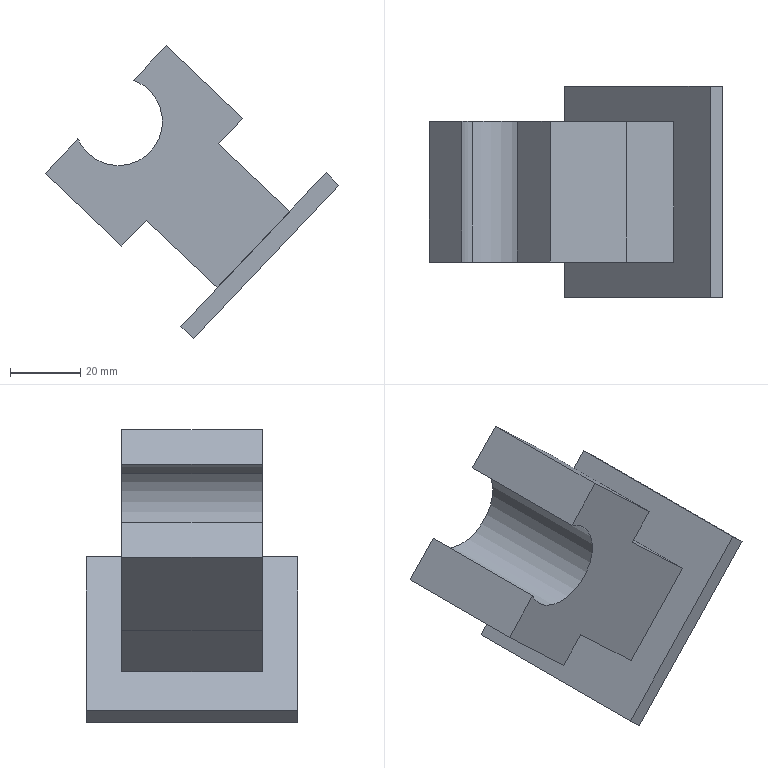Component | SolidWorks | 20mL - Glass Syringe-1_InjectionFixture-1 | 1 solid | 19 faces | box 83.45 x 60 x 83.15 mm | volume 96732 mm3 | plane 16 | cylinder 3 | commonest cylinder face diameters 25 x3
build123d program:
from build123d import *

# Parameters (mm, degrees)
BOSS_EXTRUDE1_START = -20
BOSS_EXTRUDE1_DEPTH = 40
BOSS_EXTRUDE2_DEPTH = 40
SKETCH4_W           = 60
SKETCH4_H           = 60
BOSS_EXTRUDE3_DEPTH = 5


with BuildPart() as part:
    # Sketch2 → Boss-Extrude1 (new body)
    with BuildSketch(Plane.XY.offset(BOSS_EXTRUDE1_START)):
        with BuildLine():
            Line((-21.937, -5), (-11.456, -5))
            ThreePointArc((-11.456, -5), (0, 12.5), (11.456, -5))
            Line((11.456, -5), (21.937, -5))
            ThreePointArc((21.937, -5), (0, 22.5), (-21.937, -5))
        make_face()
    extrude(amount=-BOSS_EXTRUDE1_DEPTH)

    # Sketch3 → Boss-Extrude2 (add)
    with BuildSketch(Plane.XY.offset(-20)):
        Polygon((15, 25.844), (15, 52.844), (-15, 52.844), (-15, 25.844), (-15, 25), (-25, 25), (-25, 20), (-25, -5), (-21.937, -5), (-17.95, 2.034), (-12.785, 12.264), (2.398, 17.259), (11.226, 13.398), (21.937, -5), (25, -5), (25, 20), (25, 25), (15, 25), align=None)
    extrude(amount=-BOSS_EXTRUDE2_DEPTH)

    # Sketch4 → Boss-Extrude3 (add)
    with BuildSketch(Plane(origin=(0, 52.844, 0), x_dir=(1, 0, 0), z_dir=(0, 1, 0))):
        with Locations((0, 40)):
            Rectangle(SKETCH4_W, SKETCH4_H)
    extrude(amount=BOSS_EXTRUDE3_DEPTH)


solid = part.part

# Placed as in the assembly
solid = solid.moved(Location((417.806, 1252, -1928.012), (90, 0, -133.462)))
STEP:
#1=CARTESIAN_POINT('',(15.996,50.079,-76.098));
#2=VERTEX_POINT('',#1);
#3=CARTESIAN_POINT('',(16.111,50.079,-76.263));
#4=VERTEX_POINT('',#3);
#5=CARTESIAN_POINT('',(16.449,50.079,-75.906));
#6=DIRECTION('',(0.,-1.,0.));
#7=DIRECTION('',(0.6879,0.,0.7258));
#8=AXIS2_PLACEMENT_3D('',#5,#6,#7);
#9=CIRCLE('',#8,0.4921);
#10=EDGE_CURVE('',#2,#4,#9,.T.);
#11=ORIENTED_EDGE('',*,*,#10,.T.);
#12=CARTESIAN_POINT('',(16.111,51.654,-76.263));
#13=VERTEX_POINT('',#12);
#14=CARTESIAN_POINT('',(16.111,50.079,-76.263));
#15=DIRECTION('',(-0.,1.,-0.));
#16=VECTOR('',#15,39.37);
#17=LINE('',#14,#16);
#18=EDGE_CURVE('',#4,#13,#17,.T.);
#19=ORIENTED_EDGE('',*,*,#18,.T.);
#20=CARTESIAN_POINT('',(15.996,51.654,-76.098));
#21=VERTEX_POINT('',#20);
#22=CARTESIAN_POINT('',(16.449,51.654,-75.906));
#23=DIRECTION('',(0.,-1.,0.));
#24=DIRECTION('',(0.6879,0.,0.7258));
#25=AXIS2_PLACEMENT_3D('',#22,#23,#24);
#26=CIRCLE('',#25,0.4921);
#27=EDGE_CURVE('',#21,#13,#26,.T.);
#28=ORIENTED_EDGE('',*,*,#27,.F.);
#29=CARTESIAN_POINT('',(15.996,50.079,-76.098));
#30=DIRECTION('',(-0.,1.,-0.));
#31=VECTOR('',#30,39.37);
#32=LINE('',#29,#31);
#33=EDGE_CURVE('',#2,#21,#32,.T.);
#34=ORIENTED_EDGE('',*,*,#33,.F.);
#35=EDGE_LOOP('',(#11,#19,#28,#34));
#36=FACE_OUTER_BOUND('',#35,.T.);
#37=CARTESIAN_POINT('',(16.449,50.079,-75.906));
#38=DIRECTION('',(-0.,1.,-0.));
#39=DIRECTION('',(0.6879,0.,0.7258));
#40=AXIS2_PLACEMENT_3D('',#37,#38,#39);
#41=CYLINDRICAL_SURFACE('',#40,0.4921);
#42=ADVANCED_FACE('',(#36),#41,.F.);
#43=ORIENTED_EDGE('',*,*,#18,.F.);
#44=CARTESIAN_POINT('',(16.788,50.079,-75.549));
#45=VERTEX_POINT('',#44);
#46=CARTESIAN_POINT('',(16.449,50.079,-75.906));
#47=DIRECTION('',(0.,-1.,0.));
#48=DIRECTION('',(0.6879,0.,0.7258));
#49=AXIS2_PLACEMENT_3D('',#46,#47,#48);
#50=CIRCLE('',#49,0.4921);
#51=EDGE_CURVE('',#4,#45,#50,.T.);
#52=ORIENTED_EDGE('',*,*,#51,.T.);
#53=CARTESIAN_POINT('',(16.788,51.654,-75.549));
#54=VERTEX_POINT('',#53);
#55=CARTESIAN_POINT('',(16.788,50.079,-75.549));
#56=DIRECTION('',(-0.,1.,-0.));
#57=VECTOR('',#56,39.37);
#58=LINE('',#55,#57);
#59=EDGE_CURVE('',#45,#54,#58,.T.);
#60=ORIENTED_EDGE('',*,*,#59,.T.);
#61=CARTESIAN_POINT('',(16.449,51.654,-75.906));
#62=DIRECTION('',(0.,-1.,0.));
#63=DIRECTION('',(0.6879,0.,0.7258));
#64=AXIS2_PLACEMENT_3D('',#61,#62,#63);
#65=CIRCLE('',#64,0.4921);
#66=EDGE_CURVE('',#13,#54,#65,.T.);
#67=ORIENTED_EDGE('',*,*,#66,.F.);
#68=EDGE_LOOP('',(#43,#52,#60,#67));
#69=FACE_OUTER_BOUND('',#68,.T.);
#70=CARTESIAN_POINT('',(16.449,50.079,-75.906));
#71=DIRECTION('',(-0.,1.,-0.));
#72=DIRECTION('',(0.6879,0.,0.7258));
#73=AXIS2_PLACEMENT_3D('',#70,#71,#72);
#74=CYLINDRICAL_SURFACE('',#73,0.4921);
#75=ADVANCED_FACE('',(#69),#74,.F.);
#76=CARTESIAN_POINT('',(16.616,51.654,-75.443));
#77=VERTEX_POINT('',#76);
#78=CARTESIAN_POINT('',(16.983,51.654,-75.056));
#79=VERTEX_POINT('',#78);
#80=CARTESIAN_POINT('',(16.616,51.654,-75.443));
#81=DIRECTION('',(0.6879,0.,0.7258));
#82=VECTOR('',#81,39.37);
#83=LINE('',#80,#82);
#84=EDGE_CURVE('',#77,#79,#83,.T.);
#85=ORIENTED_EDGE('',*,*,#84,.F.);
#86=CARTESIAN_POINT('',(16.616,50.079,-75.443));
#87=VERTEX_POINT('',#86);
#88=CARTESIAN_POINT('',(16.616,50.079,-75.443));
#89=DIRECTION('',(-0.,1.,-0.));
#90=VECTOR('',#89,39.37);
#91=LINE('',#88,#90);
#92=EDGE_CURVE('',#87,#77,#91,.T.);
#93=ORIENTED_EDGE('',*,*,#92,.F.);
#94=CARTESIAN_POINT('',(16.983,50.079,-75.056));
#95=VERTEX_POINT('',#94);
#96=CARTESIAN_POINT('',(16.616,50.079,-75.443));
#97=DIRECTION('',(0.6879,0.,0.7258));
#98=VECTOR('',#97,39.37);
#99=LINE('',#96,#98);
#100=EDGE_CURVE('',#87,#95,#99,.T.);
#101=ORIENTED_EDGE('',*,*,#100,.T.);
#102=CARTESIAN_POINT('',(16.983,50.079,-75.056));
#103=DIRECTION('',(-0.,1.,-0.));
#104=VECTOR('',#103,39.37);
#105=LINE('',#102,#104);
#106=EDGE_CURVE('',#95,#79,#105,.T.);
#107=ORIENTED_EDGE('',*,*,#106,.T.);
#108=EDGE_LOOP('',(#85,#93,#101,#107));
#109=FACE_OUTER_BOUND('',#108,.T.);
#110=CARTESIAN_POINT('',(16.616,50.079,-75.443));
#111=DIRECTION('',(-0.7258,-0.,0.6879));
#112=DIRECTION('',(0.,-1.,0.));
#113=AXIS2_PLACEMENT_3D('',#110,#111,#112);
#114=PLANE('',#113);
#115=ADVANCED_FACE('',(#109),#114,.T.);
#116=ORIENTED_EDGE('',*,*,#59,.F.);
#117=CARTESIAN_POINT('',(16.449,50.079,-75.906));
#118=DIRECTION('',(0.,-1.,0.));
#119=DIRECTION('',(0.6879,0.,0.7258));
#120=AXIS2_PLACEMENT_3D('',#117,#118,#119);
#121=CIRCLE('',#120,0.4921);
#122=EDGE_CURVE('',#45,#87,#121,.T.);
#123=ORIENTED_EDGE('',*,*,#122,.T.);
#124=ORIENTED_EDGE('',*,*,#92,.T.);
#125=CARTESIAN_POINT('',(16.449,51.654,-75.906));
#126=DIRECTION('',(0.,-1.,0.));
#127=DIRECTION('',(0.6879,0.,0.7258));
#128=AXIS2_PLACEMENT_3D('',#125,#126,#127);
#129=CIRCLE('',#128,0.4921);
#130=EDGE_CURVE('',#54,#77,#129,.T.);
#131=ORIENTED_EDGE('',*,*,#130,.F.);
#132=EDGE_LOOP('',(#116,#123,#124,#131));
#133=FACE_OUTER_BOUND('',#132,.T.);
#134=CARTESIAN_POINT('',(16.449,50.079,-75.906));
#135=DIRECTION('',(-0.,1.,-0.));
#136=DIRECTION('',(0.6879,0.,0.7258));
#137=AXIS2_PLACEMENT_3D('',#134,#135,#136);
#138=CYLINDRICAL_SURFACE('',#137,0.4921);
#139=ADVANCED_FACE('',(#133),#138,.F.);
#140=CARTESIAN_POINT('',(15.629,51.654,-76.485));
#141=VERTEX_POINT('',#140);
#142=CARTESIAN_POINT('',(15.712,51.654,-76.397));
#143=DIRECTION('',(0.6879,0.,0.7258));
#144=VECTOR('',#143,39.37);
#145=LINE('',#142,#144);
#146=EDGE_CURVE('',#141,#21,#145,.T.);
#147=ORIENTED_EDGE('',*,*,#146,.F.);
#148=CARTESIAN_POINT('',(15.629,50.079,-76.485));
#149=VERTEX_POINT('',#148);
#150=CARTESIAN_POINT('',(15.629,50.079,-76.485));
#151=DIRECTION('',(-0.,1.,-0.));
#152=VECTOR('',#151,39.37);
#153=LINE('',#150,#152);
#154=EDGE_CURVE('',#149,#141,#153,.T.);
#155=ORIENTED_EDGE('',*,*,#154,.F.);
#156=CARTESIAN_POINT('',(15.712,50.079,-76.397));
#157=DIRECTION('',(0.6879,0.,0.7258));
#158=VECTOR('',#157,39.37);
#159=LINE('',#156,#158);
#160=EDGE_CURVE('',#149,#2,#159,.T.);
#161=ORIENTED_EDGE('',*,*,#160,.T.);
#162=ORIENTED_EDGE('',*,*,#33,.T.);
#163=EDGE_LOOP('',(#147,#155,#161,#162));
#164=FACE_OUTER_BOUND('',#163,.T.);
#165=CARTESIAN_POINT('',(15.712,50.079,-76.397));
#166=DIRECTION('',(-0.7258,-0.,0.6879));
#167=DIRECTION('',(0.,-1.,0.));
#168=AXIS2_PLACEMENT_3D('',#165,#166,#167);
#169=PLANE('',#168);
#170=ADVANCED_FACE('',(#164),#169,.T.);
#171=ORIENTED_EDGE('',*,*,#160,.F.);
#172=CARTESIAN_POINT('',(16.486,50.079,-77.297));
#173=VERTEX_POINT('',#172);
#174=CARTESIAN_POINT('',(16.486,50.079,-77.297));
#175=DIRECTION('',(-0.7258,-0.,0.6879));
#176=VECTOR('',#175,39.37);
#177=LINE('',#174,#176);
#178=EDGE_CURVE('',#173,#149,#177,.T.);
#179=ORIENTED_EDGE('',*,*,#178,.F.);
#180=CARTESIAN_POINT('',(16.757,50.079,-77.012));
#181=VERTEX_POINT('',#180);
#182=CARTESIAN_POINT('',(16.486,50.079,-77.297));
#183=DIRECTION('',(-0.6879,-0.,-0.7258));
#184=VECTOR('',#183,39.37);
#185=LINE('',#182,#184);
#186=EDGE_CURVE('',#181,#173,#185,.T.);
#187=ORIENTED_EDGE('',*,*,#186,.F.);
#188=CARTESIAN_POINT('',(17.553,50.079,-77.766));
#189=VERTEX_POINT('',#188);
#190=CARTESIAN_POINT('',(17.553,50.079,-77.766));
#191=DIRECTION('',(-0.7258,-0.,0.6879));
#192=VECTOR('',#191,39.37);
#193=LINE('',#190,#192);
#194=EDGE_CURVE('',#189,#181,#193,.T.);
#195=ORIENTED_EDGE('',*,*,#194,.F.);
#196=CARTESIAN_POINT('',(18.365,50.079,-76.908));
#197=VERTEX_POINT('',#196);
#198=CARTESIAN_POINT('',(18.365,50.079,-76.908));
#199=DIRECTION('',(-0.6879,-0.,-0.7258));
#200=VECTOR('',#199,39.37);
#201=LINE('',#198,#200);
#202=EDGE_CURVE('',#197,#189,#201,.T.);
#203=ORIENTED_EDGE('',*,*,#202,.F.);
#204=CARTESIAN_POINT('',(17.57,50.079,-76.154));
#205=VERTEX_POINT('',#204);
#206=CARTESIAN_POINT('',(17.594,50.079,-76.177));
#207=DIRECTION('',(0.7258,0.,-0.6879));
#208=VECTOR('',#207,39.37);
#209=LINE('',#206,#208);
#210=EDGE_CURVE('',#205,#197,#209,.T.);
#211=ORIENTED_EDGE('',*,*,#210,.F.);
#212=CARTESIAN_POINT('',(17.84,50.079,-75.869));
#213=VERTEX_POINT('',#212);
#214=CARTESIAN_POINT('',(17.57,50.079,-76.154));
#215=DIRECTION('',(-0.6879,-0.,-0.7258));
#216=VECTOR('',#215,39.37);
#217=LINE('',#214,#216);
#218=EDGE_CURVE('',#213,#205,#217,.T.);
#219=ORIENTED_EDGE('',*,*,#218,.F.);
#220=CARTESIAN_POINT('',(16.983,50.079,-75.056));
#221=DIRECTION('',(0.7258,0.,-0.6879));
#222=VECTOR('',#221,39.37);
#223=LINE('',#220,#222);
#224=EDGE_CURVE('',#95,#213,#223,.T.);
#225=ORIENTED_EDGE('',*,*,#224,.F.);
#226=ORIENTED_EDGE('',*,*,#100,.F.);
#227=ORIENTED_EDGE('',*,*,#122,.F.);
#228=ORIENTED_EDGE('',*,*,#51,.F.);
#229=ORIENTED_EDGE('',*,*,#10,.F.);
#230=EDGE_LOOP('',(#171,#179,#187,#195,#203,#211,#219,#225,#226,#227,#228,#229));
#231=FACE_OUTER_BOUND('',#230,.T.);
#232=CARTESIAN_POINT('',(16.449,50.079,-75.906));
#233=DIRECTION('',(-0.,1.,-0.));
#234=DIRECTION('',(0.6879,0.,0.7258));
#235=AXIS2_PLACEMENT_3D('',#232,#233,#234);
#236=PLANE('',#235);
#237=ADVANCED_FACE('',(#231),#236,.F.);
#238=ORIENTED_EDGE('',*,*,#84,.T.);
#239=CARTESIAN_POINT('',(17.84,51.654,-75.869));
#240=VERTEX_POINT('',#239);
#241=CARTESIAN_POINT('',(17.84,51.654,-75.869));
#242=DIRECTION('',(0.7258,0.,-0.6879));
#243=VECTOR('',#242,39.37);
#244=LINE('',#241,#243);
#245=EDGE_CURVE('',#79,#240,#244,.T.);
#246=ORIENTED_EDGE('',*,*,#245,.T.);
#247=CARTESIAN_POINT('',(17.57,51.654,-76.154));
#248=VERTEX_POINT('',#247);
#249=CARTESIAN_POINT('',(17.57,51.654,-76.154));
#250=DIRECTION('',(-0.6879,-0.,-0.7258));
#251=VECTOR('',#250,39.37);
#252=LINE('',#249,#251);
#253=EDGE_CURVE('',#240,#248,#252,.T.);
#254=ORIENTED_EDGE('',*,*,#253,.T.);
#255=CARTESIAN_POINT('',(18.365,51.654,-76.908));
#256=VERTEX_POINT('',#255);
#257=CARTESIAN_POINT('',(17.594,51.654,-76.177));
#258=DIRECTION('',(0.7258,0.,-0.6879));
#259=VECTOR('',#258,39.37);
#260=LINE('',#257,#259);
#261=EDGE_CURVE('',#248,#256,#260,.T.);
#262=ORIENTED_EDGE('',*,*,#261,.T.);
#263=CARTESIAN_POINT('',(17.553,51.654,-77.766));
#264=VERTEX_POINT('',#263);
#265=CARTESIAN_POINT('',(18.365,51.654,-76.908));
#266=DIRECTION('',(-0.6879,-0.,-0.7258));
#267=VECTOR('',#266,39.37);
#268=LINE('',#265,#267);
#269=EDGE_CURVE('',#256,#264,#268,.T.);
#270=ORIENTED_EDGE('',*,*,#269,.T.);
#271=CARTESIAN_POINT('',(16.757,51.654,-77.012));
#272=VERTEX_POINT('',#271);
#273=CARTESIAN_POINT('',(16.781,51.654,-77.035));
#274=DIRECTION('',(-0.7258,-0.,0.6879));
#275=VECTOR('',#274,39.37);
#276=LINE('',#273,#275);
#277=EDGE_CURVE('',#264,#272,#276,.T.);
#278=ORIENTED_EDGE('',*,*,#277,.T.);
#279=CARTESIAN_POINT('',(16.486,51.654,-77.297));
#280=VERTEX_POINT('',#279);
#281=CARTESIAN_POINT('',(16.486,51.654,-77.297));
#282=DIRECTION('',(-0.6879,-0.,-0.7258));
#283=VECTOR('',#282,39.37);
#284=LINE('',#281,#283);
#285=EDGE_CURVE('',#272,#280,#284,.T.);
#286=ORIENTED_EDGE('',*,*,#285,.T.);
#287=CARTESIAN_POINT('',(15.629,51.654,-76.485));
#288=DIRECTION('',(-0.7258,-0.,0.6879));
#289=VECTOR('',#288,39.37);
#290=LINE('',#287,#289);
#291=EDGE_CURVE('',#280,#141,#290,.T.);
#292=ORIENTED_EDGE('',*,*,#291,.T.);
#293=ORIENTED_EDGE('',*,*,#146,.T.);
#294=ORIENTED_EDGE('',*,*,#27,.T.);
#295=ORIENTED_EDGE('',*,*,#66,.T.);
#296=ORIENTED_EDGE('',*,*,#130,.T.);
#297=EDGE_LOOP('',(#238,#246,#254,#262,#270,#278,#286,#292,#293,#294,#295,#296));
#298=FACE_OUTER_BOUND('',#297,.T.);
#299=CARTESIAN_POINT('',(16.449,51.654,-75.906));
#300=DIRECTION('',(-0.,1.,-0.));
#301=DIRECTION('',(0.6879,0.,0.7258));
#302=AXIS2_PLACEMENT_3D('',#299,#300,#301);
#303=PLANE('',#302);
#304=ADVANCED_FACE('',(#298),#303,.T.);
#305=ORIENTED_EDGE('',*,*,#291,.F.);
#306=CARTESIAN_POINT('',(16.486,50.079,-77.297));
#307=DIRECTION('',(-0.,1.,-0.));
#308=VECTOR('',#307,39.37);
#309=LINE('',#306,#308);
#310=EDGE_CURVE('',#173,#280,#309,.T.);
#311=ORIENTED_EDGE('',*,*,#310,.F.);
#312=ORIENTED_EDGE('',*,*,#178,.T.);
#313=ORIENTED_EDGE('',*,*,#154,.T.);
#314=EDGE_LOOP('',(#305,#311,#312,#313));
#315=FACE_OUTER_BOUND('',#314,.T.);
#316=CARTESIAN_POINT('',(15.629,50.079,-76.485));
#317=DIRECTION('',(-0.6879,-0.,-0.7258));
#318=DIRECTION('',(-0.,1.,-0.));
#319=AXIS2_PLACEMENT_3D('',#316,#317,#318);
#320=PLANE('',#319);
#321=ADVANCED_FACE('',(#315),#320,.T.);
#322=ORIENTED_EDGE('',*,*,#285,.F.);
#323=CARTESIAN_POINT('',(16.757,50.079,-77.012));
#324=DIRECTION('',(-0.,1.,-0.));
#325=VECTOR('',#324,39.37);
#326=LINE('',#323,#325);
#327=EDGE_CURVE('',#181,#272,#326,.T.);
#328=ORIENTED_EDGE('',*,*,#327,.F.);
#329=ORIENTED_EDGE('',*,*,#186,.T.);
#330=ORIENTED_EDGE('',*,*,#310,.T.);
#331=EDGE_LOOP('',(#322,#328,#329,#330));
#332=FACE_OUTER_BOUND('',#331,.T.);
#333=CARTESIAN_POINT('',(16.486,50.079,-77.297));
#334=DIRECTION('',(0.7258,0.,-0.6879));
#335=DIRECTION('',(-0.,1.,-0.));
#336=AXIS2_PLACEMENT_3D('',#333,#334,#335);
#337=PLANE('',#336);
#338=ADVANCED_FACE('',(#332),#337,.T.);
#339=ORIENTED_EDGE('',*,*,#277,.F.);
#340=CARTESIAN_POINT('',(17.553,50.079,-77.766));
#341=DIRECTION('',(-0.,1.,-0.));
#342=VECTOR('',#341,39.37);
#343=LINE('',#340,#342);
#344=EDGE_CURVE('',#189,#264,#343,.T.);
#345=ORIENTED_EDGE('',*,*,#344,.F.);
#346=ORIENTED_EDGE('',*,*,#194,.T.);
#347=ORIENTED_EDGE('',*,*,#327,.T.);
#348=EDGE_LOOP('',(#339,#345,#346,#347));
#349=FACE_OUTER_BOUND('',#348,.T.);
#350=CARTESIAN_POINT('',(16.781,50.079,-77.035));
#351=DIRECTION('',(-0.6879,-0.,-0.7258));
#352=DIRECTION('',(-0.,1.,-0.));
#353=AXIS2_PLACEMENT_3D('',#350,#351,#352);
#354=PLANE('',#353);
#355=ADVANCED_FACE('',(#349),#354,.T.);
#356=ORIENTED_EDGE('',*,*,#261,.F.);
#357=CARTESIAN_POINT('',(17.57,50.079,-76.154));
#358=DIRECTION('',(-0.,1.,-0.));
#359=VECTOR('',#358,39.37);
#360=LINE('',#357,#359);
#361=EDGE_CURVE('',#205,#248,#360,.T.);
#362=ORIENTED_EDGE('',*,*,#361,.F.);
#363=ORIENTED_EDGE('',*,*,#210,.T.);
#364=CARTESIAN_POINT('',(18.365,50.079,-76.908));
#365=DIRECTION('',(-0.,1.,-0.));
#366=VECTOR('',#365,39.37);
#367=LINE('',#364,#366);
#368=EDGE_CURVE('',#197,#256,#367,.T.);
#369=ORIENTED_EDGE('',*,*,#368,.T.);
#370=EDGE_LOOP('',(#356,#362,#363,#369));
#371=FACE_OUTER_BOUND('',#370,.T.);
#372=CARTESIAN_POINT('',(17.594,50.079,-76.177));
#373=DIRECTION('',(0.6879,0.,0.7258));
#374=DIRECTION('',(0.,-1.,0.));
#375=AXIS2_PLACEMENT_3D('',#372,#373,#374);
#376=PLANE('',#375);
#377=ADVANCED_FACE('',(#371),#376,.T.);
#378=ORIENTED_EDGE('',*,*,#253,.F.);
#379=CARTESIAN_POINT('',(17.84,50.079,-75.869));
#380=DIRECTION('',(-0.,1.,-0.));
#381=VECTOR('',#380,39.37);
#382=LINE('',#379,#381);
#383=EDGE_CURVE('',#213,#240,#382,.T.);
#384=ORIENTED_EDGE('',*,*,#383,.F.);
#385=ORIENTED_EDGE('',*,*,#218,.T.);
#386=ORIENTED_EDGE('',*,*,#361,.T.);
#387=EDGE_LOOP('',(#378,#384,#385,#386));
#388=FACE_OUTER_BOUND('',#387,.T.);
#389=CARTESIAN_POINT('',(17.57,50.079,-76.154));
#390=DIRECTION('',(0.7258,0.,-0.6879));
#391=DIRECTION('',(-0.,1.,-0.));
#392=AXIS2_PLACEMENT_3D('',#389,#390,#391);
#393=PLANE('',#392);
#394=ADVANCED_FACE('',(#388),#393,.T.);
#395=ORIENTED_EDGE('',*,*,#245,.F.);
#396=ORIENTED_EDGE('',*,*,#106,.F.);
#397=ORIENTED_EDGE('',*,*,#224,.T.);
#398=ORIENTED_EDGE('',*,*,#383,.T.);
#399=EDGE_LOOP('',(#395,#396,#397,#398));
#400=FACE_OUTER_BOUND('',#399,.T.);
#401=CARTESIAN_POINT('',(17.84,50.079,-75.869));
#402=DIRECTION('',(0.6879,0.,0.7258));
#403=DIRECTION('',(0.,-1.,0.));
#404=AXIS2_PLACEMENT_3D('',#401,#402,#403);
#405=PLANE('',#404);
#406=ADVANCED_FACE('',(#400),#405,.T.);
#407=CARTESIAN_POINT('',(17.147,49.685,-78.194));
#408=VERTEX_POINT('',#407);
#409=CARTESIAN_POINT('',(17.147,52.047,-78.194));
#410=VERTEX_POINT('',#409);
#411=CARTESIAN_POINT('',(17.147,49.685,-78.194));
#412=DIRECTION('',(-0.,1.,-0.));
#413=VECTOR('',#412,39.37);
#414=LINE('',#411,#413);
#415=EDGE_CURVE('',#408,#410,#414,.T.);
#416=ORIENTED_EDGE('',*,*,#415,.F.);
#417=CARTESIAN_POINT('',(18.772,49.685,-76.48));
#418=VERTEX_POINT('',#417);
#419=CARTESIAN_POINT('',(18.772,49.685,-76.48));
#420=DIRECTION('',(-0.6879,-0.,-0.7258));
#421=VECTOR('',#420,39.37);
#422=LINE('',#419,#421);
#423=EDGE_CURVE('',#418,#408,#422,.T.);
#424=ORIENTED_EDGE('',*,*,#423,.F.);
#425=CARTESIAN_POINT('',(18.772,52.047,-76.48));
#426=VERTEX_POINT('',#425);
#427=CARTESIAN_POINT('',(18.772,49.685,-76.48));
#428=DIRECTION('',(0.,-1.,0.));
#429=VECTOR('',#428,39.37);
#430=LINE('',#427,#429);
#431=EDGE_CURVE('',#426,#418,#430,.T.);
#432=ORIENTED_EDGE('',*,*,#431,.F.);
#433=CARTESIAN_POINT('',(18.772,52.047,-76.48));
#434=DIRECTION('',(0.6879,0.,0.7258));
#435=VECTOR('',#434,39.37);
#436=LINE('',#433,#435);
#437=EDGE_CURVE('',#410,#426,#436,.T.);
#438=ORIENTED_EDGE('',*,*,#437,.F.);
#439=EDGE_LOOP('',(#416,#424,#432,#438));
#440=FACE_OUTER_BOUND('',#439,.T.);
#441=ORIENTED_EDGE('',*,*,#269,.F.);
#442=ORIENTED_EDGE('',*,*,#368,.F.);
#443=ORIENTED_EDGE('',*,*,#202,.T.);
#444=ORIENTED_EDGE('',*,*,#344,.T.);
#445=EDGE_LOOP('',(#441,#442,#443,#444));
#446=FACE_BOUND('',#445,.T.);
#447=CARTESIAN_POINT('',(17.959,52.441,-77.337));
#448=DIRECTION('',(-0.7258,-0.,0.6879));
#449=DIRECTION('',(0.6879,0.,0.7258));
#450=AXIS2_PLACEMENT_3D('',#447,#448,#449);
#451=PLANE('',#450);
#452=ADVANCED_FACE('',(#440,#446),#451,.T.);
#453=ORIENTED_EDGE('',*,*,#415,.T.);
#454=CARTESIAN_POINT('',(17.29,52.047,-78.33));
#455=VERTEX_POINT('',#454);
#456=CARTESIAN_POINT('',(17.29,52.047,-78.33));
#457=DIRECTION('',(-0.7258,-0.,0.6879));
#458=VECTOR('',#457,39.37);
#459=LINE('',#456,#458);
#460=EDGE_CURVE('',#455,#410,#459,.T.);
#461=ORIENTED_EDGE('',*,*,#460,.F.);
#462=CARTESIAN_POINT('',(17.29,49.685,-78.33));
#463=VERTEX_POINT('',#462);
#464=CARTESIAN_POINT('',(17.29,49.685,-78.33));
#465=DIRECTION('',(-0.,1.,-0.));
#466=VECTOR('',#465,39.37);
#467=LINE('',#464,#466);
#468=EDGE_CURVE('',#463,#455,#467,.T.);
#469=ORIENTED_EDGE('',*,*,#468,.F.);
#470=CARTESIAN_POINT('',(17.29,49.685,-78.33));
#471=DIRECTION('',(-0.7258,-0.,0.6879));
#472=VECTOR('',#471,39.37);
#473=LINE('',#470,#472);
#474=EDGE_CURVE('',#463,#408,#473,.T.);
#475=ORIENTED_EDGE('',*,*,#474,.T.);
#476=EDGE_LOOP('',(#453,#461,#469,#475));
#477=FACE_OUTER_BOUND('',#476,.T.);
#478=CARTESIAN_POINT('',(17.29,49.685,-78.33));
#479=DIRECTION('',(0.6879,0.,0.7258));
#480=DIRECTION('',(0.7258,0.,-0.6879));
#481=AXIS2_PLACEMENT_3D('',#478,#479,#480);
#482=PLANE('',#481);
#483=ADVANCED_FACE('',(#477),#482,.F.);
#484=ORIENTED_EDGE('',*,*,#437,.T.);
#485=CARTESIAN_POINT('',(18.914,52.047,-76.615));
#486=VERTEX_POINT('',#485);
#487=CARTESIAN_POINT('',(18.914,52.047,-76.615));
#488=DIRECTION('',(-0.7258,-0.,0.6879));
#489=VECTOR('',#488,39.37);
#490=LINE('',#487,#489);
#491=EDGE_CURVE('',#486,#426,#490,.T.);
#492=ORIENTED_EDGE('',*,*,#491,.F.);
#493=CARTESIAN_POINT('',(18.914,52.047,-76.615));
#494=DIRECTION('',(0.6879,0.,0.7258));
#495=VECTOR('',#494,39.37);
#496=LINE('',#493,#495);
#497=EDGE_CURVE('',#455,#486,#496,.T.);
#498=ORIENTED_EDGE('',*,*,#497,.F.);
#499=ORIENTED_EDGE('',*,*,#460,.T.);
#500=EDGE_LOOP('',(#484,#492,#498,#499));
#501=FACE_OUTER_BOUND('',#500,.T.);
#502=CARTESIAN_POINT('',(18.914,52.047,-76.615));
#503=DIRECTION('',(0.,-1.,0.));
#504=DIRECTION('',(-0.6879,-0.,-0.7258));
#505=AXIS2_PLACEMENT_3D('',#502,#503,#504);
#506=PLANE('',#505);
#507=ADVANCED_FACE('',(#501),#506,.F.);
#508=ORIENTED_EDGE('',*,*,#431,.T.);
#509=CARTESIAN_POINT('',(18.914,49.685,-76.615));
#510=VERTEX_POINT('',#509);
#511=CARTESIAN_POINT('',(18.914,49.685,-76.615));
#512=DIRECTION('',(-0.7258,-0.,0.6879));
#513=VECTOR('',#512,39.37);
#514=LINE('',#511,#513);
#515=EDGE_CURVE('',#510,#418,#514,.T.);
#516=ORIENTED_EDGE('',*,*,#515,.F.);
#517=CARTESIAN_POINT('',(18.914,49.685,-76.615));
#518=DIRECTION('',(0.,-1.,0.));
#519=VECTOR('',#518,39.37);
#520=LINE('',#517,#519);
#521=EDGE_CURVE('',#486,#510,#520,.T.);
#522=ORIENTED_EDGE('',*,*,#521,.F.);
#523=ORIENTED_EDGE('',*,*,#491,.T.);
#524=EDGE_LOOP('',(#508,#516,#522,#523));
#525=FACE_OUTER_BOUND('',#524,.T.);
#526=CARTESIAN_POINT('',(18.914,49.685,-76.615));
#527=DIRECTION('',(-0.6879,-0.,-0.7258));
#528=DIRECTION('',(-0.7258,-0.,0.6879));
#529=AXIS2_PLACEMENT_3D('',#526,#527,#528);
#530=PLANE('',#529);
#531=ADVANCED_FACE('',(#525),#530,.F.);
#532=ORIENTED_EDGE('',*,*,#423,.T.);
#533=ORIENTED_EDGE('',*,*,#474,.F.);
#534=CARTESIAN_POINT('',(18.914,49.685,-76.615));
#535=DIRECTION('',(-0.6879,-0.,-0.7258));
#536=VECTOR('',#535,39.37);
#537=LINE('',#534,#536);
#538=EDGE_CURVE('',#510,#463,#537,.T.);
#539=ORIENTED_EDGE('',*,*,#538,.F.);
#540=ORIENTED_EDGE('',*,*,#515,.T.);
#541=EDGE_LOOP('',(#532,#533,#539,#540));
#542=FACE_OUTER_BOUND('',#541,.T.);
#543=CARTESIAN_POINT('',(18.914,49.685,-76.615));
#544=DIRECTION('',(-0.,1.,0.));
#545=DIRECTION('',(0.6879,0.,0.7258));
#546=AXIS2_PLACEMENT_3D('',#543,#544,#545);
#547=PLANE('',#546);
#548=ADVANCED_FACE('',(#542),#547,.F.);
#549=ORIENTED_EDGE('',*,*,#468,.T.);
#550=ORIENTED_EDGE('',*,*,#497,.T.);
#551=ORIENTED_EDGE('',*,*,#521,.T.);
#552=ORIENTED_EDGE('',*,*,#538,.T.);
#553=EDGE_LOOP('',(#549,#550,#551,#552));
#554=FACE_OUTER_BOUND('',#553,.T.);
#555=CARTESIAN_POINT('',(18.102,52.441,-77.472));
#556=DIRECTION('',(-0.7258,-0.,0.6879));
#557=DIRECTION('',(0.6879,0.,0.7258));
#558=AXIS2_PLACEMENT_3D('',#555,#556,#557);
#559=PLANE('',#558);
#560=ADVANCED_FACE('',(#554),#559,.F.);
#561=CLOSED_SHELL('',(#42,#75,#115,#139,#170,#237,#304,#321,#338,#355,#377,#394,#406,#452,#483,#507,#531,#548,#560));
#562=MANIFOLD_SOLID_BREP('',#561);
#563=CARTESIAN_POINT('',(0.,0.,0.));
#564=DIRECTION('',(0.,0.,1.));
#565=DIRECTION('',(1.,0.,0.));
#566=AXIS2_PLACEMENT_3D('',#563,#564,#565);
#567=(LENGTH_UNIT()NAMED_UNIT(*)SI_UNIT($,.METRE.));
#568=LENGTH_MEASURE_WITH_UNIT(LENGTH_MEASURE(0.0254),#567);
#569=DIMENSIONAL_EXPONENTS(1.,0.,0.,0.,0.,0.,0.);
#570=(CONVERSION_BASED_UNIT('',#568)LENGTH_UNIT()NAMED_UNIT(#569));
#571=UNCERTAINTY_MEASURE_WITH_UNIT(LENGTH_MEASURE(0.00001),#570,'','');
#572=(NAMED_UNIT(*)PLANE_ANGLE_UNIT()SI_UNIT($,.RADIAN.));
#573=(NAMED_UNIT(*)SI_UNIT($,.STERADIAN.)SOLID_ANGLE_UNIT());
#574=(GEOMETRIC_REPRESENTATION_CONTEXT(3)GLOBAL_UNCERTAINTY_ASSIGNED_CONTEXT((#571))GLOBAL_UNIT_ASSIGNED_CONTEXT((#570,#572,#573))REPRESENTATION_CONTEXT('',''));
#575=ADVANCED_BREP_SHAPE_REPRESENTATION('',(#562,#566),#574);
#576=COLOUR_RGB('',0.7922,0.8196,0.9333);
#577=FILL_AREA_STYLE_COLOUR('',#576);
#578=FILL_AREA_STYLE('',(#577));
#579=SURFACE_STYLE_FILL_AREA(#578);
#580=SURFACE_SIDE_STYLE('',(#579));
#581=SURFACE_STYLE_USAGE(.BOTH.,#580);
#582=PRESENTATION_STYLE_ASSIGNMENT((#581));
#583=STYLED_ITEM('',(#582),#562);
#584=PRESENTATION_LAYER_ASSIGNMENT('','',(#583));
#585=(LENGTH_UNIT()NAMED_UNIT(*)SI_UNIT($,.METRE.));
#586=LENGTH_MEASURE_WITH_UNIT(LENGTH_MEASURE(0.0254),#585);
#587=DIMENSIONAL_EXPONENTS(1.,0.,0.,0.,0.,0.,0.);
#588=(CONVERSION_BASED_UNIT('',#586)LENGTH_UNIT()NAMED_UNIT(#587));
#589=UNCERTAINTY_MEASURE_WITH_UNIT(LENGTH_MEASURE(0.00001),#588,'','');
#590=(NAMED_UNIT(*)PLANE_ANGLE_UNIT()SI_UNIT($,.RADIAN.));
#591=(NAMED_UNIT(*)SI_UNIT($,.STERADIAN.)SOLID_ANGLE_UNIT());
#592=(GEOMETRIC_REPRESENTATION_CONTEXT(3)GLOBAL_UNCERTAINTY_ASSIGNED_CONTEXT((#589))GLOBAL_UNIT_ASSIGNED_CONTEXT((#588,#590,#591))REPRESENTATION_CONTEXT('',''));
#593=MECHANICAL_DESIGN_GEOMETRIC_PRESENTATION_REPRESENTATION('',(#583),#592);